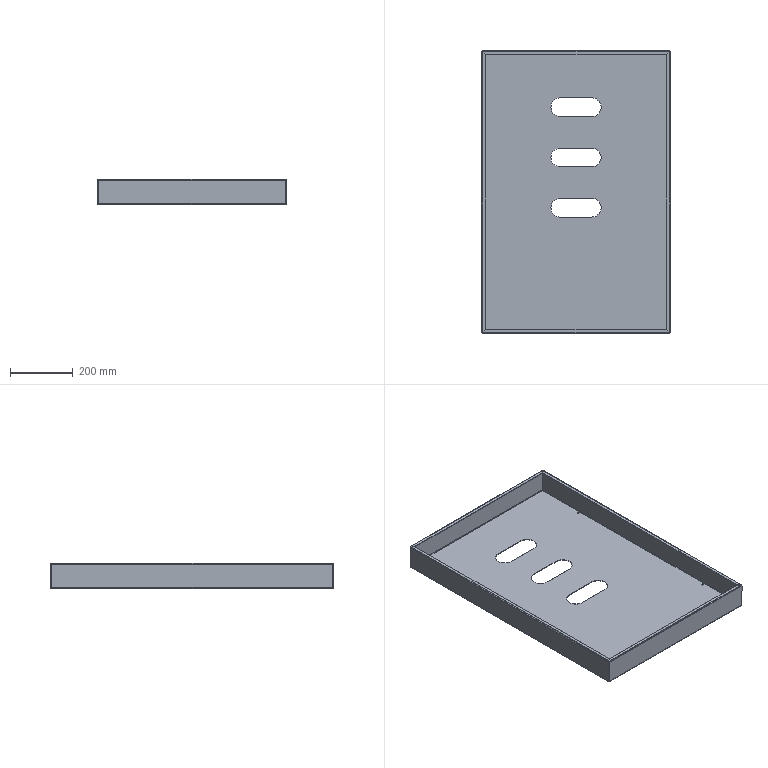Component | SolidWorks | LowerSeat-1 | 1 solid | 93 faces | volume 1540682 mm3 | plane 44 | cylinder 33 | spline 16 | commonest cylinder face diameters 6 x16 60 x9 2 x8